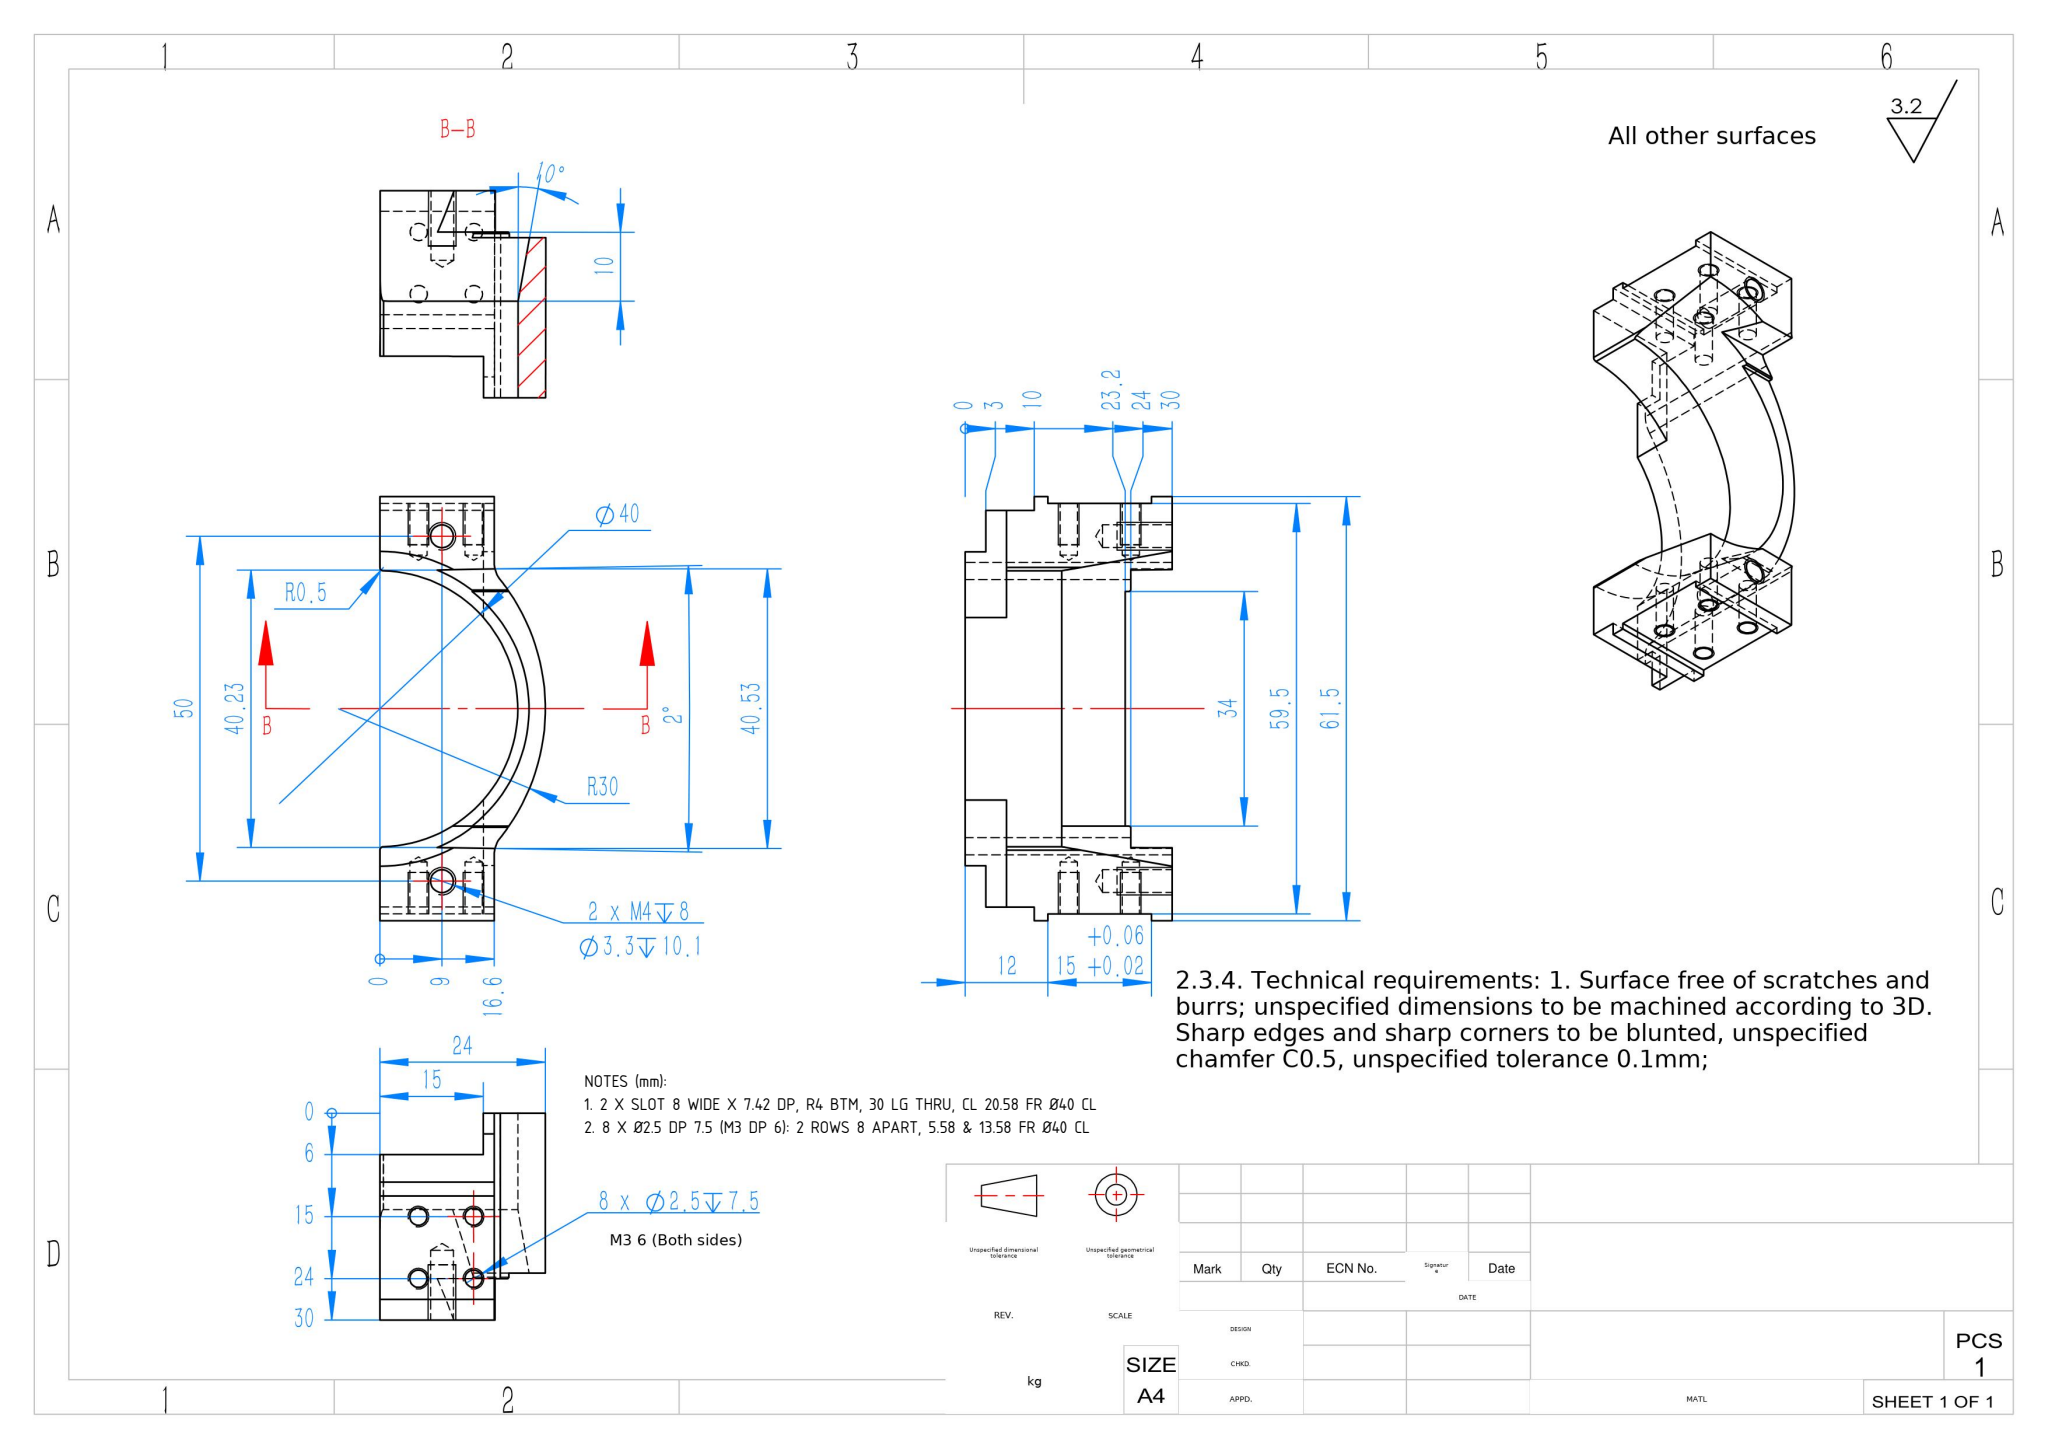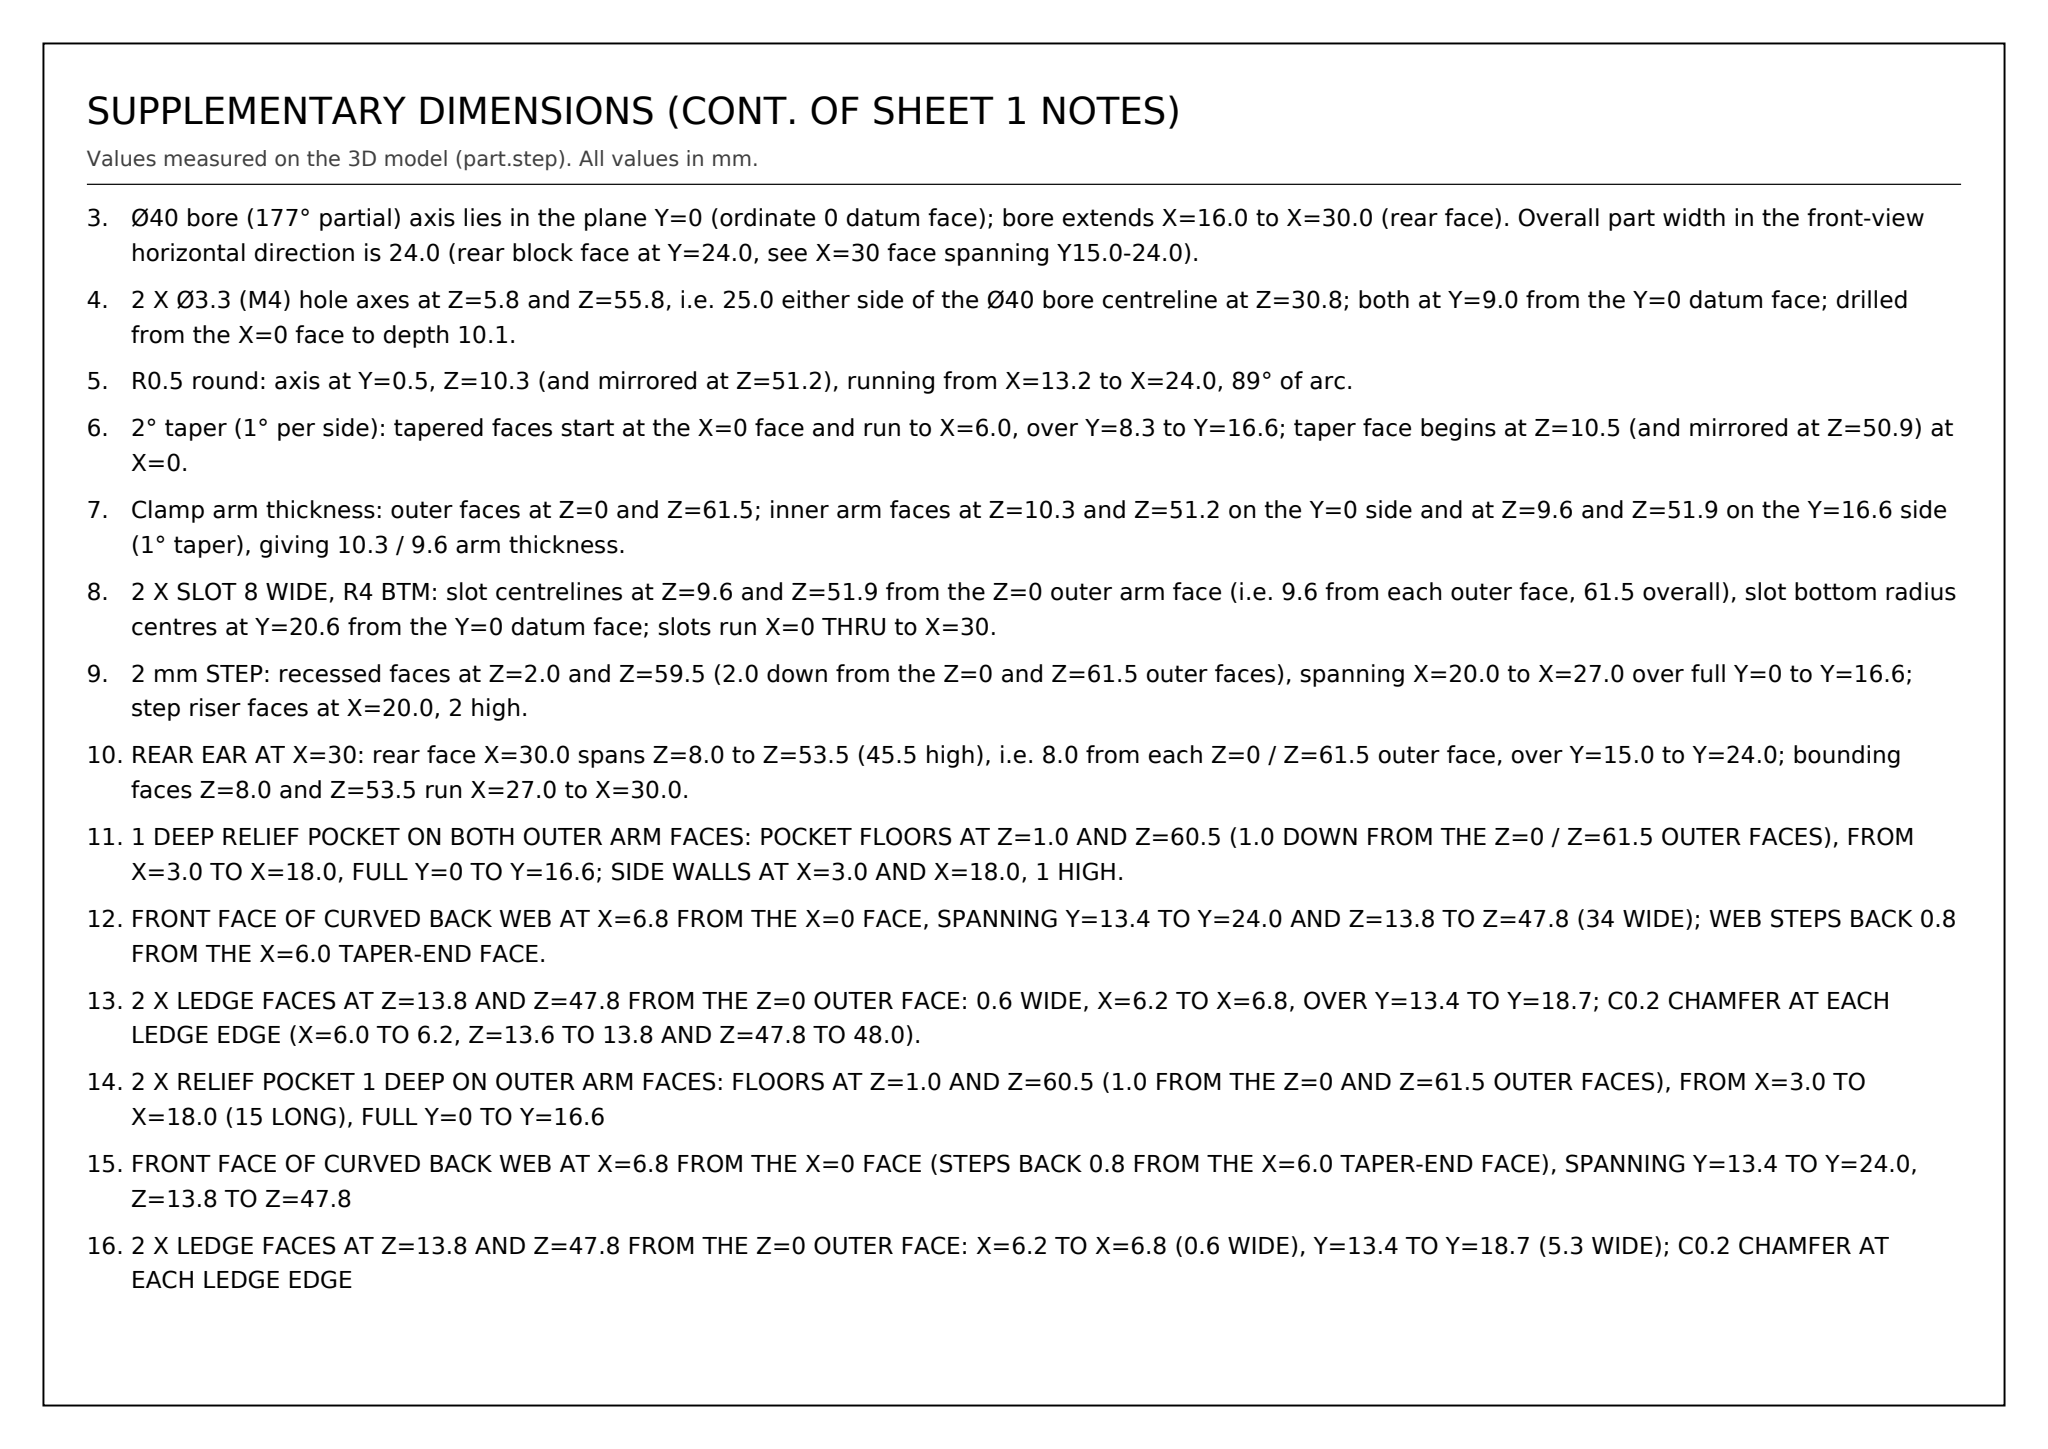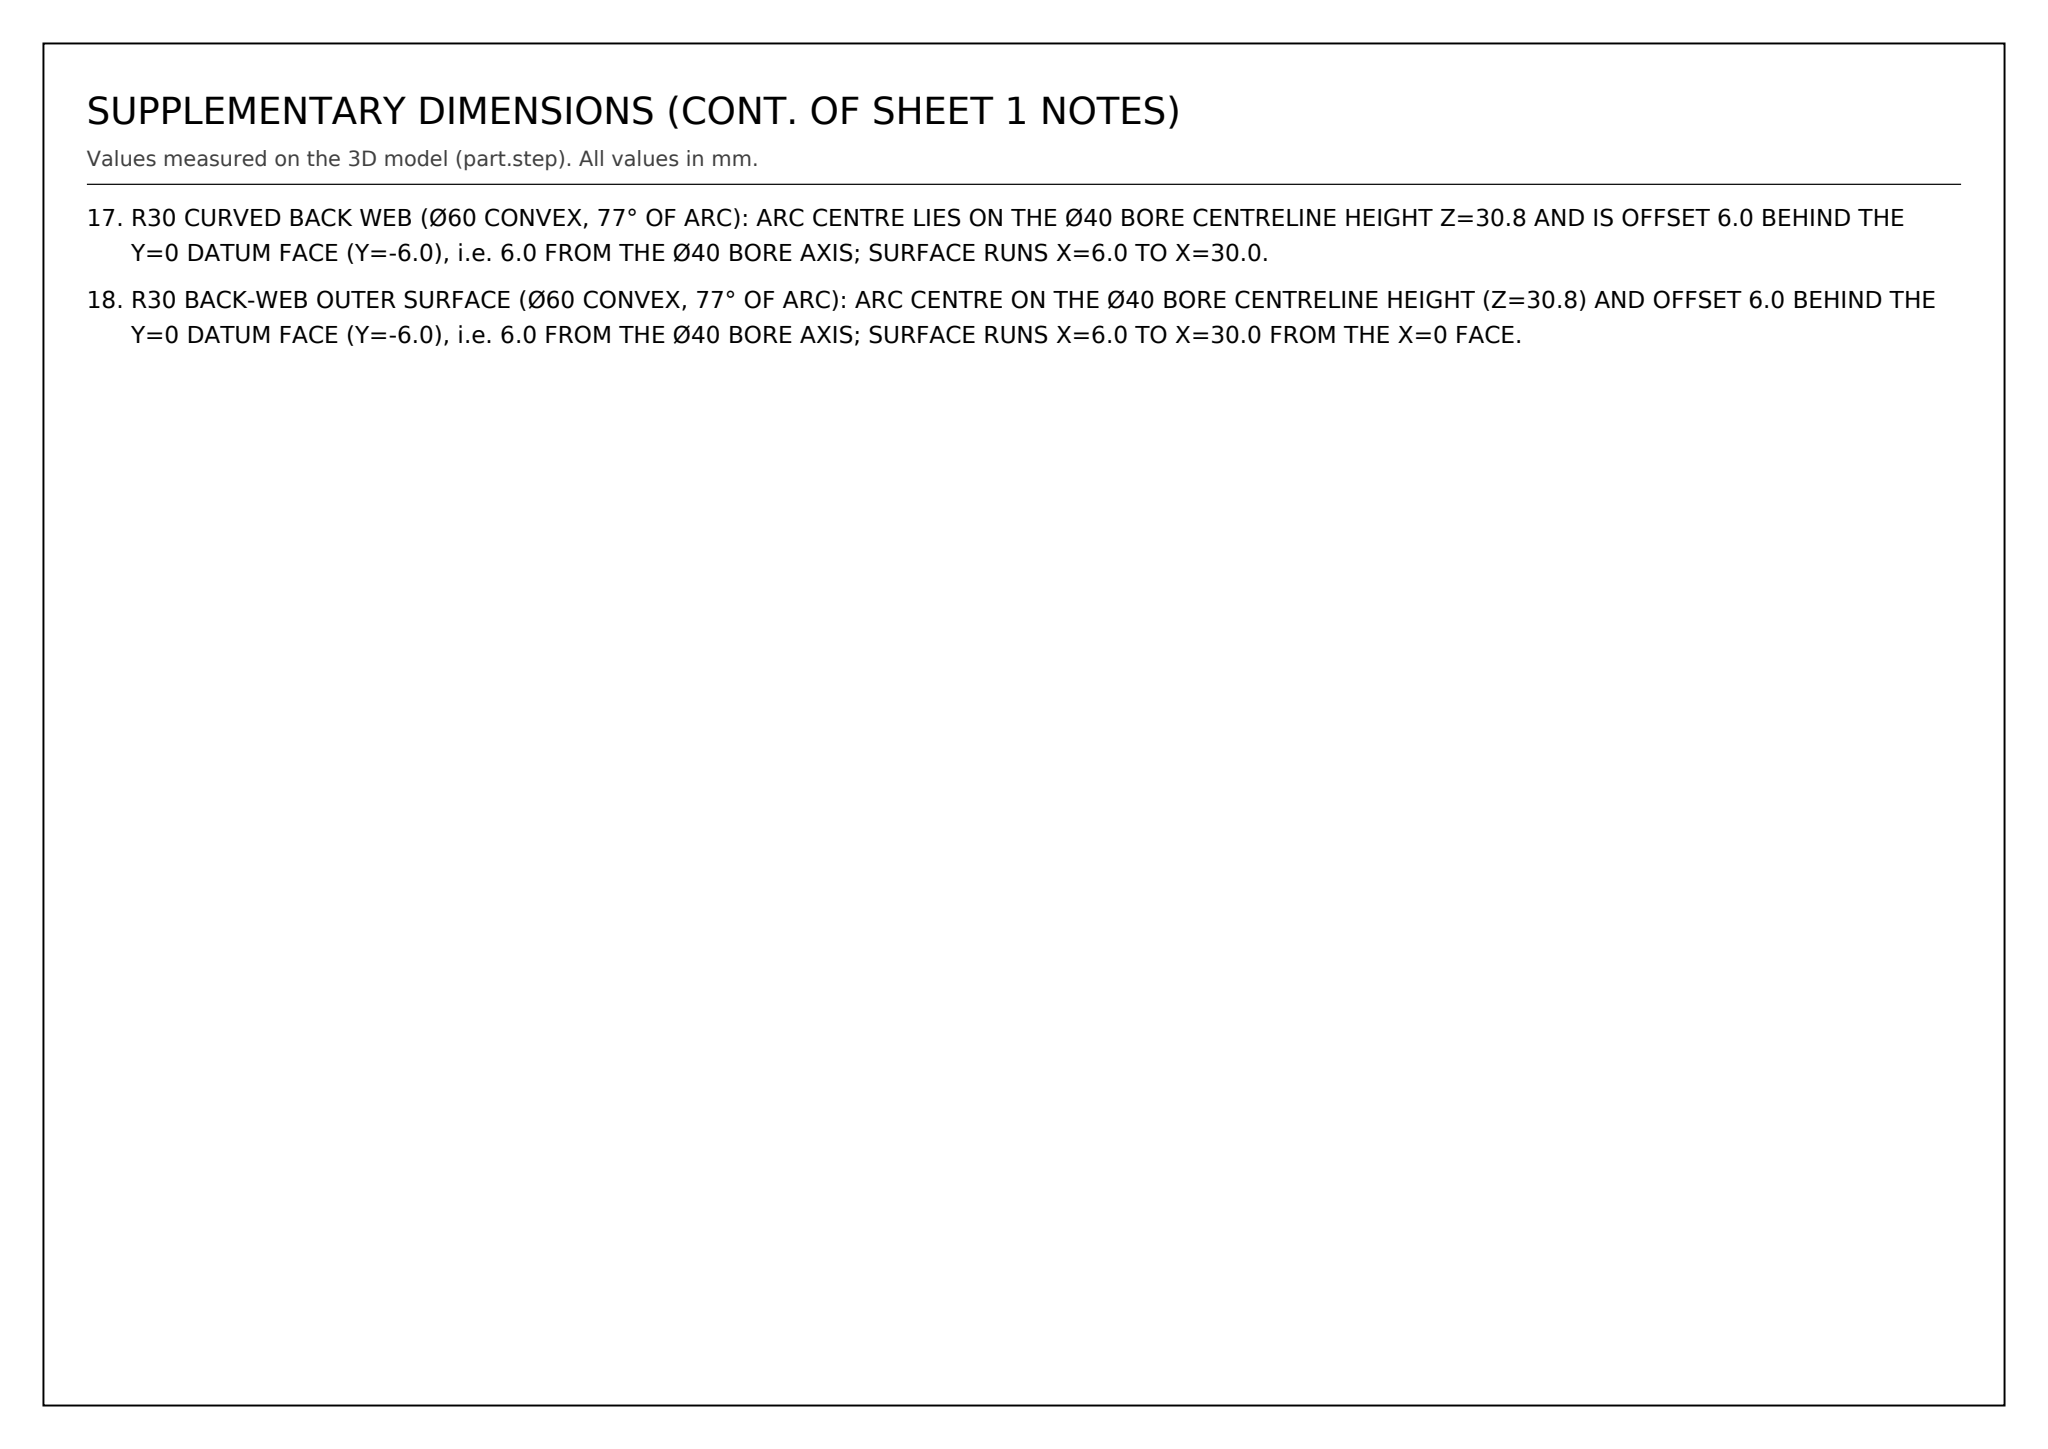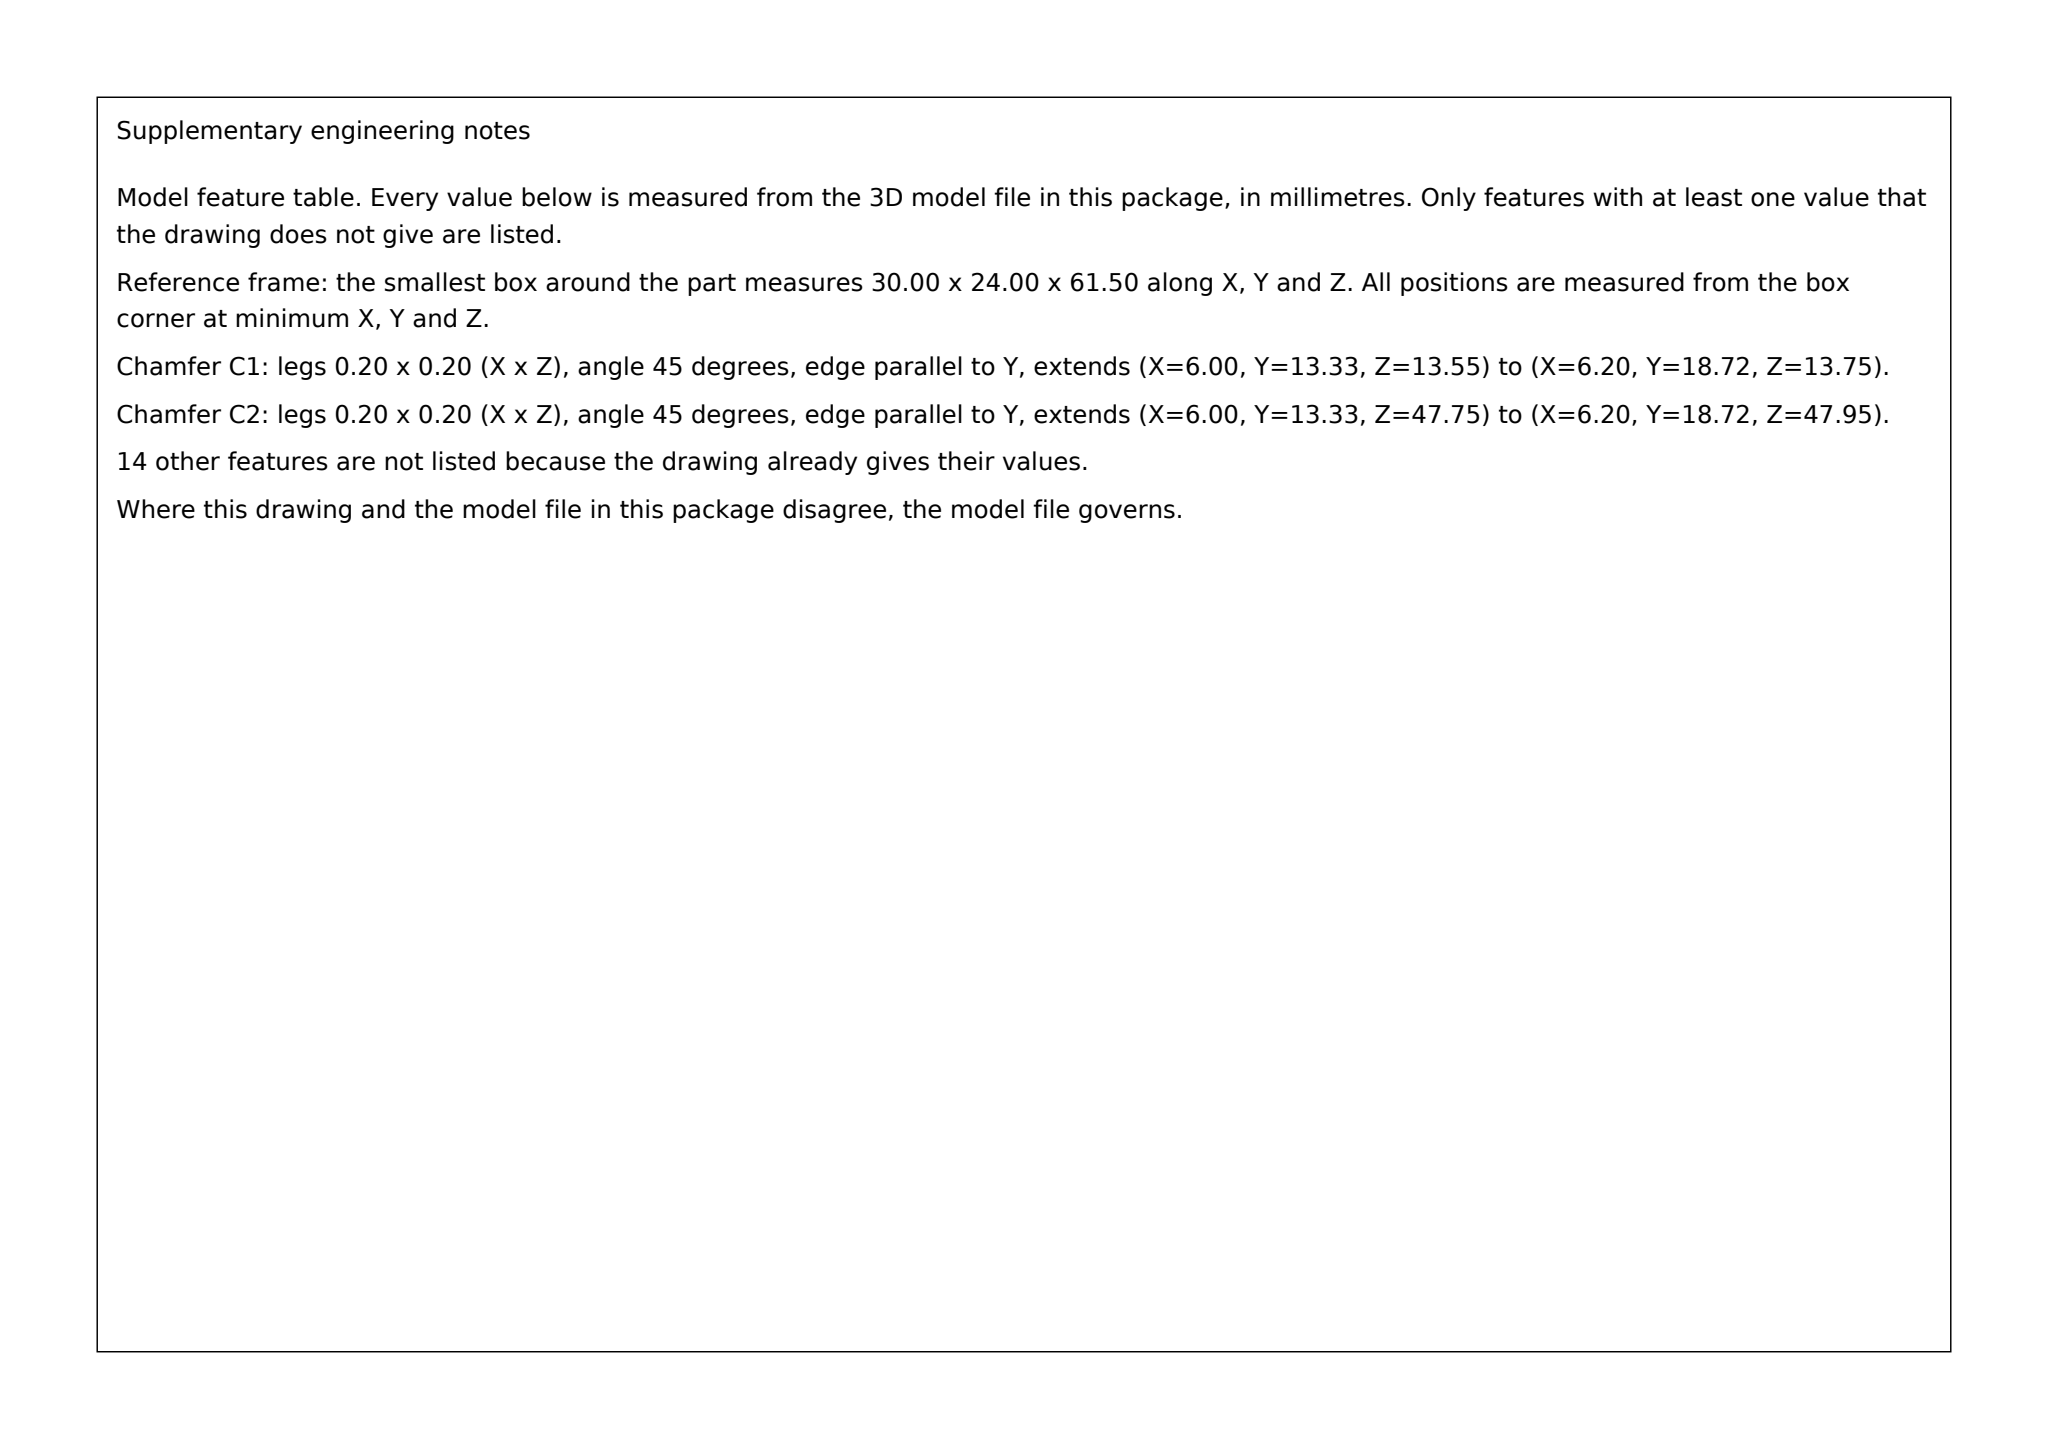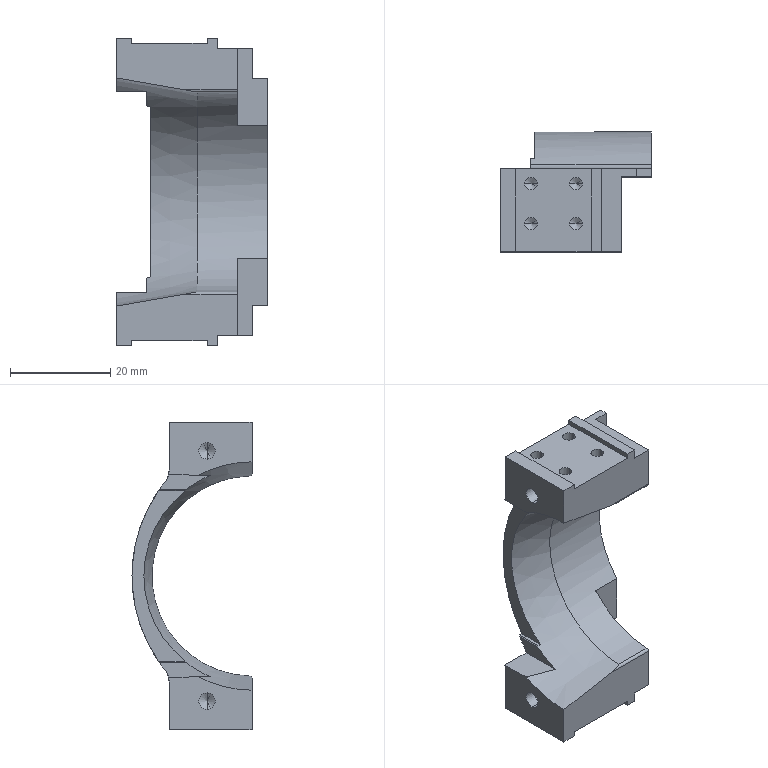Part | SolidWorks | mm | 1 solid | 86 faces | box 30 x 24 x 61.5 mm | volume 11858 mm3 | plane 38 | cylinder 26 | cone 22 | commonest cylinder face diameters 2.5 x16 3.3 x4 1 x2 8 x2 40 x1 60 x1
Drawing notes:
2 X SLOT 8 WIDE X 7.42 DP, R4 BTM, 30 LG THRU, CL 20.58 FR Ø40 CL | from the solid: Ø8 x-axis cylinders, length 30, at y=20.58, z=9.55 & 51.95; break out at y=24.001 face -> depth 24.001-16.58=7.42, plane y=16.58
8 X Ø2.5 DP 7.5 (M3 DP 6): 2 ROWS 8 APART, 5.58 & 13.58 FR Ø40 CL | from the solid: Ø2.5 z-axis holes at y=5.58 and y=13.58 (x=6 and 15), spacing 13.58-5.58=8.0; Ø40 bore axis at y=0
Ø40 bore (177° partial) axis lies in the plane Y=0 (ordinate 0 datum face); bore extends X=16.0 to X=30.0 (rear face). Overall part width in the front-view horizontal direction is 24.0 (rear block face at Y=24.0, see X=30 face spanning Y15.0-24.0). | from the solid: cylinders: concave arc dia 40.0, axis x, axis_pos [y=0.0, z=30.8], from 16.0 to 30.0; axis_planes x=30 extent y[15.0,24.0]; bbox_xyz [30.001,24.001,61.501]
2 X Ø3.3 (M4) hole axes at Z=5.8 and Z=55.8, i.e. 25.0 either side of the Ø40 bore centreline at Z=30.8; both at Y=9.0 from the Y=0 datum face; drilled from the X=0 face to depth 10.1. | from the solid: cylinders: hole/bore dia 3.3, axis x, axis_pos [y=9.0, z=5.8] and [y=9.0, z=55.8], from 0.0 to 10.1; Ø40 bore axis z=30.8
R0.5 round: axis at Y=0.5, Z=10.3 (and mirrored at Z=51.2), running from X=13.2 to X=24.0, 89° of arc. | from the solid: cylinders: convex arc (round/outer radius) dia 1.0, axis x, axis_pos [y=0.5, z=10.3] and [y=0.5, z=51.2], from 13.2 to 24.0, arc 89
2° taper (1° per side): tapered faces start at the X=0 face and run to X=6.0, over Y=8.3 to Y=16.6; taper face begins at Z=10.5 (and mirrored at Z=50.9) at X=0. | from the solid: inclined_planes: angle_to_xyz_axes [90,89,1], bbox_from [0.0,8.3,10.5] and [0.0,8.3,50.9], size [6.0,8.4,0.1]
Clamp arm thickness: outer faces at Z=0 and Z=61.5; inner arm faces at Z=10.3 and Z=51.2 on the Y=0 side and at Z=9.6 and Z=51.9 on the Y=16.6 side (1° taper), giving 10.3 / 9.6 arm thickness. | from the solid: axis_planes: y=0 extent z[0.0,10.3] and z[51.2,61.5]; y=16.6 extent z[0.0,9.6] and z[51.9,61.5]
2 X SLOT 8 WIDE, R4 BTM: slot centrelines at Z=9.6 and Z=51.9 from the Z=0 outer arm face (i.e. 9.6 from each outer face, 61.5 overall), slot bottom radius centres at Y=20.6 from the Y=0 datum face; slots run X=0 THRU to X=30. | from the solid: cylinders: concave arc dia 8.0 axis x at (y=20.6, z=9.6) and (y=20.6, z=51.9), from X=0 to X=30
2 mm STEP: recessed faces at Z=2.0 and Z=59.5 (2.0 down from the Z=0 and Z=61.5 outer faces), spanning X=20.0 to X=27.0 over full Y=0 to Y=16.6; step riser faces at X=20.0, 2 high. | from the solid: axis_planes: z=2.0 and z=59.5, extent x[20.0,27.0] y[0.0,16.6]; x=20.0, extent z[0.0,2.0] and z[59.5,61.5]
REAR EAR AT X=30: rear face X=30.0 spans Z=8.0 to Z=53.5 (45.5 high), i.e. 8.0 from each Z=0 / Z=61.5 outer face, over Y=15.0 to Y=24.0; bounding faces Z=8.0 and Z=53.5 run X=27.0 to X=30.0. | from the solid: axis_planes: x=30.0 extent y[15.0,24.0] z[8.0,53.5]; z=8.0 and z=53.5 extent x[27.0,30.0] y[15.0,16.6]
1 DEEP RELIEF POCKET ON BOTH OUTER ARM FACES: POCKET FLOORS AT Z=1.0 AND Z=60.5 (1.0 DOWN FROM THE Z=0 / Z=61.5 OUTER FACES), FROM X=3.0 TO X=18.0, FULL Y=0 TO Y=16.6; SIDE WALLS AT X=3.0 AND X=18.0, 1 HIGH. | from the solid: axis_planes z=1.0 and z=60.5 extent x[3.0,18.0] y[0.0,16.6]; axis_planes x=3.0 and x=18.0 extent z[0.0,1.0] and z[60.5,61.5]
FRONT FACE OF CURVED BACK WEB AT X=6.8 FROM THE X=0 FACE, SPANNING Y=13.4 TO Y=24.0 AND Z=13.8 TO Z=47.8 (34 WIDE); WEB STEPS BACK 0.8 FROM THE X=6.0 TAPER-END FACE. | from the solid: axis_plane x=6.8 extent y[13.4,24.0] z[13.8,47.8]; axis_plane x=6.0 extent y[8.3,18.6]
2 X LEDGE FACES AT Z=13.8 AND Z=47.8 FROM THE Z=0 OUTER FACE: 0.6 WIDE, X=6.2 TO X=6.8, OVER Y=13.4 TO Y=18.7; C0.2 CHAMFER AT EACH LEDGE EDGE (X=6.0 TO 6.2, Z=13.6 TO 13.8 AND Z=47.8 TO 48.0). | from the solid: axis_planes z=13.8 and z=47.8 extent x[6.2,6.8] y[13.4,18.7]; inclined_planes 45/90/45 at [6.0,13.3,13.6] and [6.0,13.3,47.8] size 0.2x5.4x0.2
2 X RELIEF POCKET 1 DEEP ON OUTER ARM FACES: FLOORS AT Z=1.0 AND Z=60.5 (1.0 FROM THE Z=0 AND Z=61.5 OUTER FACES), FROM X=3.0 TO X=18.0 (15 LONG), FULL Y=0 TO Y=16.6 | from the solid: axis_planes z=1.0 and z=60.5 extent x[3.0,18.0] y[0,16.6]; walls x=3.0 and x=18.0 with z extents [0,1.0] and [60.5,61.5]
FRONT FACE OF CURVED BACK WEB AT X=6.8 FROM THE X=0 FACE (STEPS BACK 0.8 FROM THE X=6.0 TAPER-END FACE), SPANNING Y=13.4 TO Y=24.0, Z=13.8 TO Z=47.8 | from the solid: axis_plane x=6.8 extent y[13.4,24.0] z[13.8,47.8]; axis_plane x=6.0 taper-end faces
2 X LEDGE FACES AT Z=13.8 AND Z=47.8 FROM THE Z=0 OUTER FACE: X=6.2 TO X=6.8 (0.6 WIDE), Y=13.4 TO Y=18.7 (5.3 WIDE); C0.2 CHAMFER AT EACH LEDGE EDGE | from the solid: axis_planes z=13.8 and z=47.8 extent x[6.2,6.8] y[13.4,18.7]; inclined_planes 45° at [6.0,13.3,13.6] and [6.0,13.3,47.8] size 0.2x5.4x0.2
R30 CURVED BACK WEB (Ø60 CONVEX, 77° OF ARC): ARC CENTRE LIES ON THE Ø40 BORE CENTRELINE HEIGHT Z=30.8 AND IS OFFSET 6.0 BEHIND THE Y=0 DATUM FACE (Y=-6.0), i.e. 6.0 FROM THE Ø40 BORE AXIS; SURFACE RUNS X=6.0 TO X=30.0. | from the solid: cylinders: convex arc (round/outer radius) dia 60.0, axis x, axis_pos_other_axes [null, -6.0, 30.8], from 6.0 to 30.0, arc_deg 77; Ø40 bore axis at [null, 0.0, 30.8]
R30 BACK-WEB OUTER SURFACE (Ø60 CONVEX, 77° OF ARC): ARC CENTRE ON THE Ø40 BORE CENTRELINE HEIGHT (Z=30.8) AND OFFSET 6.0 BEHIND THE Y=0 DATUM FACE (Y=-6.0), i.e. 6.0 FROM THE Ø40 BORE AXIS; SURFACE RUNS X=6.0 TO X=30.0 FROM THE X=0 FACE. | from the solid: cylinders: convex arc (round/outer radius), dia 60.0, axis x at (y=-6.0, z=30.8), from x=6.0 to x=30.0, arc_deg 77